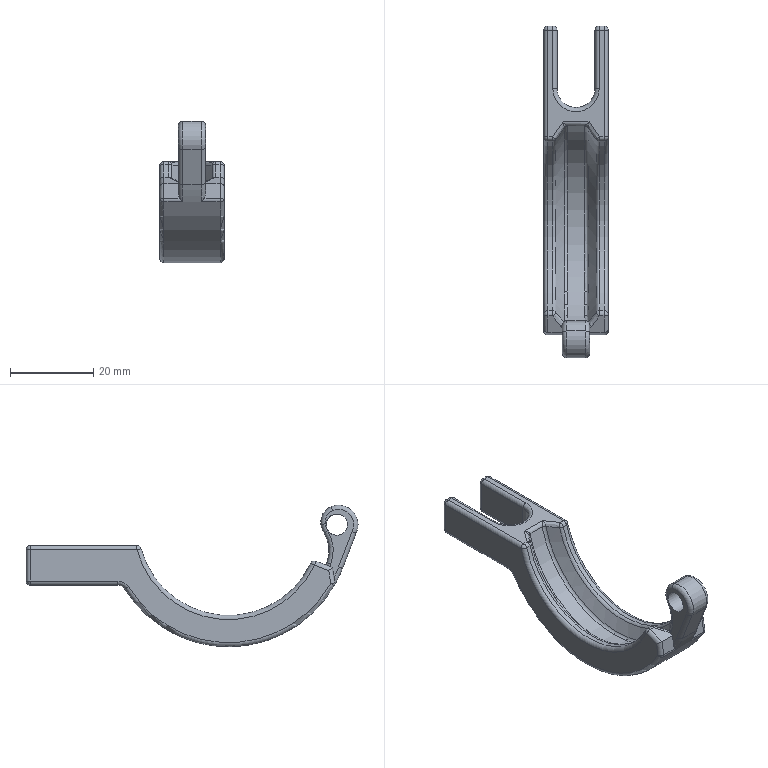Component | NX | LOWER_CLASP | 1 solid | 109 faces | volume 7804 mm3 | cylinder 40 | torus 24 | sphere 18 | plane 15 | spline 10 | cone 2 | commonest cylinder face diameters 2 x29 43.5 x2 58.5 x1 9.1 x1 4 x1 50.5 x1 9.322 x1 5.1 x1